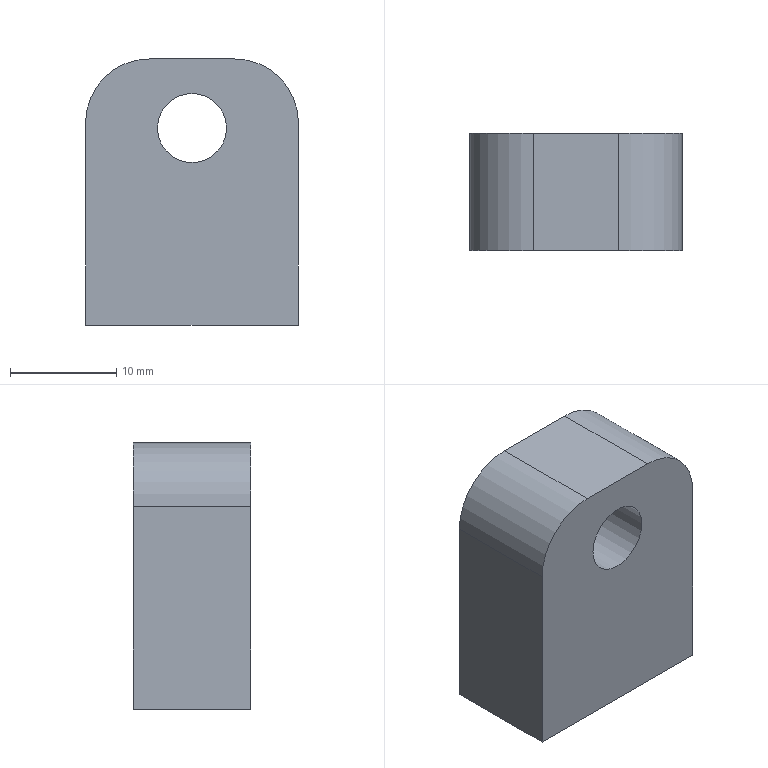Component | NX | SMALL_BRACKET | 1 solid | 13 faces | box 20 x 11 x 25 mm | volume 4714 mm3 | plane 8 | cylinder 5 | commonest cylinder face diameters 12 x2 4 x2 6.5 x1
STEP:
#1=CARTESIAN_POINT('',(0.,0.,0.));
#2=DIRECTION('',(0.,0.,1.));
#3=DIRECTION('',(1.,0.,0.));
#4=AXIS2_PLACEMENT_3D('',#1,#2,#3);
#5=CARTESIAN_POINT('',(9.,19.,36.5));
#6=VERTEX_POINT('',#5);
#7=CARTESIAN_POINT('',(9.,19.,17.5));
#8=VERTEX_POINT('',#7);
#9=CARTESIAN_POINT('',(9.,19.,42.5));
#10=DIRECTION('',(0.,0.,-1.));
#11=VECTOR('',#10,1.);
#12=LINE('',#9,#11);
#13=CARTESIAN_POINT('',(9.,19.,42.5));
#14=DIRECTION('',(1.,0.,0.));
#15=DIRECTION('',(0.,0.,1.));
#16=AXIS2_PLACEMENT_3D('',#13,#14,#15);
#17=PLANE('',#16);
#18=CARTESIAN_POINT('',(0.,0.));
#19=DIRECTION('',(-1.,0.));
#20=VECTOR('',#19,1.);
#21=LINE('',#18,#20);
#22=(GEOMETRIC_REPRESENTATION_CONTEXT(2)PARAMETRIC_REPRESENTATION_CONTEXT()REPRESENTATION_CONTEXT('',''));
#23=DEFINITIONAL_REPRESENTATION('',(#21),#22);
#24=PCURVE('',#17,#23);
#25=CARTESIAN_POINT('',(19.,19.,36.));
#26=DIRECTION('',(0.,-1.,0.));
#27=DIRECTION('',(0.,0.,-1.));
#28=AXIS2_PLACEMENT_3D('',#25,#26,#27);
#29=PLANE('',#28);
#30=CARTESIAN_POINT('',(-6.5,-10.));
#31=DIRECTION('',(1.,0.));
#32=VECTOR('',#31,1.);
#33=LINE('',#30,#32);
#34=(GEOMETRIC_REPRESENTATION_CONTEXT(2)PARAMETRIC_REPRESENTATION_CONTEXT()REPRESENTATION_CONTEXT('',''));
#35=DEFINITIONAL_REPRESENTATION('',(#33),#34);
#36=PCURVE('',#29,#35);
#37=SURFACE_CURVE('',#12,(#24,#36),.PCURVE_S1.);
#38=EDGE_CURVE('',#6,#8,#37,.T.);
#39=ORIENTED_EDGE('',*,*,#38,.F.);
#40=CARTESIAN_POINT('',(9.,30.,36.5));
#41=VERTEX_POINT('',#40);
#42=CARTESIAN_POINT('',(9.,19.,36.5));
#43=DIRECTION('',(0.,1.,0.));
#44=VECTOR('',#43,1.);
#45=LINE('',#42,#44);
#46=CARTESIAN_POINT('',(-6.,0.));
#47=DIRECTION('',(0.,-1.));
#48=VECTOR('',#47,1.);
#49=LINE('',#46,#48);
#50=(GEOMETRIC_REPRESENTATION_CONTEXT(2)PARAMETRIC_REPRESENTATION_CONTEXT()REPRESENTATION_CONTEXT('',''));
#51=DEFINITIONAL_REPRESENTATION('',(#49),#50);
#52=PCURVE('',#17,#51);
#53=CARTESIAN_POINT('',(15.,19.,36.5));
#54=DIRECTION('',(0.,1.,0.));
#55=DIRECTION('',(0.,0.,1.));
#56=AXIS2_PLACEMENT_3D('',#53,#54,#55);
#57=CYLINDRICAL_SURFACE('',#56,6.);
#58=CARTESIAN_POINT('',(4.712,0.));
#59=DIRECTION('',(0.,1.));
#60=VECTOR('',#59,1.);
#61=LINE('',#58,#60);
#62=(GEOMETRIC_REPRESENTATION_CONTEXT(2)PARAMETRIC_REPRESENTATION_CONTEXT()REPRESENTATION_CONTEXT('',''));
#63=DEFINITIONAL_REPRESENTATION('',(#61),#62);
#64=PCURVE('',#57,#63);
#65=SURFACE_CURVE('',#45,(#52,#64),.PCURVE_S1.);
#66=EDGE_CURVE('',#6,#41,#65,.T.);
#67=ORIENTED_EDGE('',*,*,#66,.T.);
#68=CARTESIAN_POINT('',(9.,30.,17.5));
#69=VERTEX_POINT('',#68);
#70=CARTESIAN_POINT('',(9.,30.,42.5));
#71=DIRECTION('',(0.,0.,-1.));
#72=VECTOR('',#71,1.);
#73=LINE('',#70,#72);
#74=CARTESIAN_POINT('',(0.,-11.));
#75=DIRECTION('',(-1.,0.));
#76=VECTOR('',#75,1.);
#77=LINE('',#74,#76);
#78=(GEOMETRIC_REPRESENTATION_CONTEXT(2)PARAMETRIC_REPRESENTATION_CONTEXT()REPRESENTATION_CONTEXT('',''));
#79=DEFINITIONAL_REPRESENTATION('',(#77),#78);
#80=PCURVE('',#17,#79);
#81=CARTESIAN_POINT('',(19.,30.,36.));
#82=DIRECTION('',(0.,-1.,0.));
#83=DIRECTION('',(0.,0.,-1.));
#84=AXIS2_PLACEMENT_3D('',#81,#82,#83);
#85=PLANE('',#84);
#86=CARTESIAN_POINT('',(-6.5,-10.));
#87=DIRECTION('',(1.,0.));
#88=VECTOR('',#87,1.);
#89=LINE('',#86,#88);
#90=(GEOMETRIC_REPRESENTATION_CONTEXT(2)PARAMETRIC_REPRESENTATION_CONTEXT()REPRESENTATION_CONTEXT('',''));
#91=DEFINITIONAL_REPRESENTATION('',(#89),#90);
#92=PCURVE('',#85,#91);
#93=SURFACE_CURVE('',#73,(#80,#92),.PCURVE_S1.);
#94=EDGE_CURVE('',#41,#69,#93,.T.);
#95=ORIENTED_EDGE('',*,*,#94,.T.);
#96=CARTESIAN_POINT('',(9.,19.,17.5));
#97=DIRECTION('',(0.,1.,0.));
#98=VECTOR('',#97,1.);
#99=LINE('',#96,#98);
#100=CARTESIAN_POINT('',(-25.,0.));
#101=DIRECTION('',(0.,-1.));
#102=VECTOR('',#101,1.);
#103=LINE('',#100,#102);
#104=(GEOMETRIC_REPRESENTATION_CONTEXT(2)PARAMETRIC_REPRESENTATION_CONTEXT()REPRESENTATION_CONTEXT('',''));
#105=DEFINITIONAL_REPRESENTATION('',(#103),#104);
#106=PCURVE('',#17,#105);
#107=CARTESIAN_POINT('',(19.,19.,17.5));
#108=DIRECTION('',(0.,0.,1.));
#109=DIRECTION('',(-1.,0.,0.));
#110=AXIS2_PLACEMENT_3D('',#107,#108,#109);
#111=PLANE('',#110);
#112=CARTESIAN_POINT('',(10.,0.));
#113=DIRECTION('',(0.,-1.));
#114=VECTOR('',#113,1.);
#115=LINE('',#112,#114);
#116=(GEOMETRIC_REPRESENTATION_CONTEXT(2)PARAMETRIC_REPRESENTATION_CONTEXT()REPRESENTATION_CONTEXT('',''));
#117=DEFINITIONAL_REPRESENTATION('',(#115),#116);
#118=PCURVE('',#111,#117);
#119=SURFACE_CURVE('',#99,(#106,#118),.PCURVE_S1.);
#120=EDGE_CURVE('',#8,#69,#119,.T.);
#121=ORIENTED_EDGE('',*,*,#120,.F.);
#122=EDGE_LOOP('',(#39,#67,#95,#121));
#123=FACE_BOUND('',#122,.T.);
#124=ADVANCED_FACE('',(#123),#17,.F.);
#125=CARTESIAN_POINT('',(14.5,24.5,17.5));
#126=VERTEX_POINT('',#125);
#127=CARTESIAN_POINT('',(12.5,24.5,17.5));
#128=DIRECTION('',(-0.,0.,-1.));
#129=DIRECTION('',(1.,0.,-0.));
#130=AXIS2_PLACEMENT_3D('',#127,#128,#129);
#131=CIRCLE('',#130,2.);
#132=CARTESIAN_POINT('',(4.5,-5.5));
#133=CARTESIAN_POINT('',(4.5,-2.036));
#134=CARTESIAN_POINT('',(7.5,-3.768));
#135=CARTESIAN_POINT('',(10.5,-5.5));
#136=CARTESIAN_POINT('',(7.5,-7.232));
#137=CARTESIAN_POINT('',(4.5,-8.964));
#138=CARTESIAN_POINT('',(4.5,-5.5));
#139=(BOUNDED_CURVE()B_SPLINE_CURVE(2,(#132,#133,#134,#135,#136,#137,#138),.UNSPECIFIED.,.T.,.F.)B_SPLINE_CURVE_WITH_KNOTS((1,2,2,2,2,1),(-2.094,0.,2.094,4.189,6.283,8.378),.UNSPECIFIED.)CURVE()GEOMETRIC_REPRESENTATION_ITEM()RATIONAL_B_SPLINE_CURVE((1.,0.5,1.,0.5,1.,0.5,1.))REPRESENTATION_ITEM(''));
#140=(GEOMETRIC_REPRESENTATION_CONTEXT(2)PARAMETRIC_REPRESENTATION_CONTEXT()REPRESENTATION_CONTEXT('',''));
#141=DEFINITIONAL_REPRESENTATION('',(#139),#140);
#142=PCURVE('',#111,#141);
#143=CARTESIAN_POINT('',(12.5,24.5,27.5));
#144=DIRECTION('',(-0.,0.,-1.));
#145=DIRECTION('',(1.,0.,-0.));
#146=AXIS2_PLACEMENT_3D('',#143,#144,#145);
#147=CYLINDRICAL_SURFACE('',#146,2.);
#148=CARTESIAN_POINT('',(0.,10.));
#149=DIRECTION('',(1.,0.));
#150=VECTOR('',#149,1.);
#151=LINE('',#148,#150);
#152=(GEOMETRIC_REPRESENTATION_CONTEXT(2)PARAMETRIC_REPRESENTATION_CONTEXT()REPRESENTATION_CONTEXT('',''));
#153=DEFINITIONAL_REPRESENTATION('',(#151),#152);
#154=PCURVE('',#147,#153);
#155=SURFACE_CURVE('',#131,(#142,#154),.PCURVE_S1.);
#156=EDGE_CURVE('',#126,#126,#155,.T.);
#157=ORIENTED_EDGE('',*,*,#156,.F.);
#158=EDGE_LOOP('',(#157));
#159=FACE_BOUND('',#158,.T.);
#160=CARTESIAN_POINT('',(23.5,24.5,17.5));
#161=VERTEX_POINT('',#160);
#162=CARTESIAN_POINT('',(25.5,24.5,17.5));
#163=DIRECTION('',(-0.,0.,-1.));
#164=DIRECTION('',(-1.,0.,0.));
#165=AXIS2_PLACEMENT_3D('',#162,#163,#164);
#166=CIRCLE('',#165,2.);
#167=CARTESIAN_POINT('',(-4.5,-5.5));
#168=CARTESIAN_POINT('',(-4.5,-8.964));
#169=CARTESIAN_POINT('',(-7.5,-7.232));
#170=CARTESIAN_POINT('',(-10.5,-5.5));
#171=CARTESIAN_POINT('',(-7.5,-3.768));
#172=CARTESIAN_POINT('',(-4.5,-2.036));
#173=CARTESIAN_POINT('',(-4.5,-5.5));
#174=(BOUNDED_CURVE()B_SPLINE_CURVE(2,(#167,#168,#169,#170,#171,#172,#173),.UNSPECIFIED.,.T.,.F.)B_SPLINE_CURVE_WITH_KNOTS((1,2,2,2,2,1),(-2.094,0.,2.094,4.189,6.283,8.378),.UNSPECIFIED.)CURVE()GEOMETRIC_REPRESENTATION_ITEM()RATIONAL_B_SPLINE_CURVE((1.,0.5,1.,0.5,1.,0.5,1.))REPRESENTATION_ITEM(''));
#175=(GEOMETRIC_REPRESENTATION_CONTEXT(2)PARAMETRIC_REPRESENTATION_CONTEXT()REPRESENTATION_CONTEXT('',''));
#176=DEFINITIONAL_REPRESENTATION('',(#174),#175);
#177=PCURVE('',#111,#176);
#178=CARTESIAN_POINT('',(25.5,24.5,27.5));
#179=DIRECTION('',(-0.,0.,-1.));
#180=DIRECTION('',(1.,0.,-0.));
#181=AXIS2_PLACEMENT_3D('',#178,#179,#180);
#182=CYLINDRICAL_SURFACE('',#181,2.);
#183=CARTESIAN_POINT('',(3.142,10.));
#184=DIRECTION('',(1.,0.));
#185=VECTOR('',#184,1.);
#186=LINE('',#183,#185);
#187=(GEOMETRIC_REPRESENTATION_CONTEXT(2)PARAMETRIC_REPRESENTATION_CONTEXT()REPRESENTATION_CONTEXT('',''));
#188=DEFINITIONAL_REPRESENTATION('',(#186),#187);
#189=PCURVE('',#182,#188);
#190=SURFACE_CURVE('',#166,(#177,#189),.PCURVE_S1.);
#191=EDGE_CURVE('',#161,#161,#190,.T.);
#192=ORIENTED_EDGE('',*,*,#191,.F.);
#193=EDGE_LOOP('',(#192));
#194=FACE_BOUND('',#193,.T.);
#195=CARTESIAN_POINT('',(29.,30.,17.5));
#196=VERTEX_POINT('',#195);
#197=CARTESIAN_POINT('',(19.,30.,17.5));
#198=DIRECTION('',(1.,0.,-0.));
#199=VECTOR('',#198,1.);
#200=LINE('',#197,#199);
#201=CARTESIAN_POINT('',(0.,-11.));
#202=DIRECTION('',(-1.,0.));
#203=VECTOR('',#202,1.);
#204=LINE('',#201,#203);
#205=(GEOMETRIC_REPRESENTATION_CONTEXT(2)PARAMETRIC_REPRESENTATION_CONTEXT()REPRESENTATION_CONTEXT('',''));
#206=DEFINITIONAL_REPRESENTATION('',(#204),#205);
#207=PCURVE('',#111,#206);
#208=CARTESIAN_POINT('',(18.5,0.));
#209=DIRECTION('',(0.,1.));
#210=VECTOR('',#209,1.);
#211=LINE('',#208,#210);
#212=(GEOMETRIC_REPRESENTATION_CONTEXT(2)PARAMETRIC_REPRESENTATION_CONTEXT()REPRESENTATION_CONTEXT('',''));
#213=DEFINITIONAL_REPRESENTATION('',(#211),#212);
#214=PCURVE('',#85,#213);
#215=SURFACE_CURVE('',#200,(#207,#214),.PCURVE_S1.);
#216=EDGE_CURVE('',#69,#196,#215,.T.);
#217=ORIENTED_EDGE('',*,*,#216,.T.);
#218=CARTESIAN_POINT('',(29.,19.,17.5));
#219=VERTEX_POINT('',#218);
#220=CARTESIAN_POINT('',(29.,19.,17.5));
#221=DIRECTION('',(0.,1.,0.));
#222=VECTOR('',#221,1.);
#223=LINE('',#220,#222);
#224=CARTESIAN_POINT('',(-10.,0.));
#225=DIRECTION('',(0.,-1.));
#226=VECTOR('',#225,1.);
#227=LINE('',#224,#226);
#228=(GEOMETRIC_REPRESENTATION_CONTEXT(2)PARAMETRIC_REPRESENTATION_CONTEXT()REPRESENTATION_CONTEXT('',''));
#229=DEFINITIONAL_REPRESENTATION('',(#227),#228);
#230=PCURVE('',#111,#229);
#231=CARTESIAN_POINT('',(29.,19.,17.5));
#232=DIRECTION('',(-1.,0.,0.));
#233=DIRECTION('',(0.,0.,-1.));
#234=AXIS2_PLACEMENT_3D('',#231,#232,#233);
#235=PLANE('',#234);
#236=CARTESIAN_POINT('',(0.,0.));
#237=DIRECTION('',(0.,-1.));
#238=VECTOR('',#237,1.);
#239=LINE('',#236,#238);
#240=(GEOMETRIC_REPRESENTATION_CONTEXT(2)PARAMETRIC_REPRESENTATION_CONTEXT()REPRESENTATION_CONTEXT('',''));
#241=DEFINITIONAL_REPRESENTATION('',(#239),#240);
#242=PCURVE('',#235,#241);
#243=SURFACE_CURVE('',#223,(#230,#242),.PCURVE_S1.);
#244=EDGE_CURVE('',#219,#196,#243,.T.);
#245=ORIENTED_EDGE('',*,*,#244,.F.);
#246=CARTESIAN_POINT('',(9.,19.,17.5));
#247=DIRECTION('',(1.,0.,0.));
#248=VECTOR('',#247,1.);
#249=LINE('',#246,#248);
#250=CARTESIAN_POINT('',(10.,0.));
#251=DIRECTION('',(-1.,0.));
#252=VECTOR('',#251,1.);
#253=LINE('',#250,#252);
#254=(GEOMETRIC_REPRESENTATION_CONTEXT(2)PARAMETRIC_REPRESENTATION_CONTEXT()REPRESENTATION_CONTEXT('',''));
#255=DEFINITIONAL_REPRESENTATION('',(#253),#254);
#256=PCURVE('',#111,#255);
#257=CARTESIAN_POINT('',(18.5,-10.));
#258=DIRECTION('',(-0.,1.));
#259=VECTOR('',#258,1.);
#260=LINE('',#257,#259);
#261=(GEOMETRIC_REPRESENTATION_CONTEXT(2)PARAMETRIC_REPRESENTATION_CONTEXT()REPRESENTATION_CONTEXT('',''));
#262=DEFINITIONAL_REPRESENTATION('',(#260),#261);
#263=PCURVE('',#29,#262);
#264=SURFACE_CURVE('',#249,(#256,#263),.PCURVE_S1.);
#265=EDGE_CURVE('',#8,#219,#264,.T.);
#266=ORIENTED_EDGE('',*,*,#265,.F.);
#267=ORIENTED_EDGE('',*,*,#120,.T.);
#268=EDGE_LOOP('',(#217,#245,#266,#267));
#269=FACE_BOUND('',#268,.T.);
#270=ADVANCED_FACE('',(#159,#194,#269),#111,.F.);
#271=CARTESIAN_POINT('',(29.,30.,36.5));
#272=VERTEX_POINT('',#271);
#273=CARTESIAN_POINT('',(29.,30.,17.5));
#274=DIRECTION('',(0.,0.,1.));
#275=VECTOR('',#274,1.);
#276=LINE('',#273,#275);
#277=CARTESIAN_POINT('',(0.,-11.));
#278=DIRECTION('',(-1.,0.));
#279=VECTOR('',#278,1.);
#280=LINE('',#277,#279);
#281=(GEOMETRIC_REPRESENTATION_CONTEXT(2)PARAMETRIC_REPRESENTATION_CONTEXT()REPRESENTATION_CONTEXT('',''));
#282=DEFINITIONAL_REPRESENTATION('',(#280),#281);
#283=PCURVE('',#235,#282);
#284=CARTESIAN_POINT('',(18.5,10.));
#285=DIRECTION('',(-1.,0.));
#286=VECTOR('',#285,1.);
#287=LINE('',#284,#286);
#288=(GEOMETRIC_REPRESENTATION_CONTEXT(2)PARAMETRIC_REPRESENTATION_CONTEXT()REPRESENTATION_CONTEXT('',''));
#289=DEFINITIONAL_REPRESENTATION('',(#287),#288);
#290=PCURVE('',#85,#289);
#291=SURFACE_CURVE('',#276,(#283,#290),.PCURVE_S1.);
#292=EDGE_CURVE('',#196,#272,#291,.T.);
#293=ORIENTED_EDGE('',*,*,#292,.T.);
#294=CARTESIAN_POINT('',(29.,19.,36.5));
#295=VERTEX_POINT('',#294);
#296=CARTESIAN_POINT('',(29.,19.,36.5));
#297=DIRECTION('',(0.,-1.,0.));
#298=VECTOR('',#297,1.);
#299=LINE('',#296,#298);
#300=CARTESIAN_POINT('',(-19.,0.));
#301=DIRECTION('',(0.,1.));
#302=VECTOR('',#301,1.);
#303=LINE('',#300,#302);
#304=(GEOMETRIC_REPRESENTATION_CONTEXT(2)PARAMETRIC_REPRESENTATION_CONTEXT()REPRESENTATION_CONTEXT('',''));
#305=DEFINITIONAL_REPRESENTATION('',(#303),#304);
#306=PCURVE('',#235,#305);
#307=CARTESIAN_POINT('',(23.,19.,36.5));
#308=DIRECTION('',(0.,1.,0.));
#309=DIRECTION('',(0.,0.,1.));
#310=AXIS2_PLACEMENT_3D('',#307,#308,#309);
#311=CYLINDRICAL_SURFACE('',#310,6.);
#312=CARTESIAN_POINT('',(1.571,0.));
#313=DIRECTION('',(0.,-1.));
#314=VECTOR('',#313,1.);
#315=LINE('',#312,#314);
#316=(GEOMETRIC_REPRESENTATION_CONTEXT(2)PARAMETRIC_REPRESENTATION_CONTEXT()REPRESENTATION_CONTEXT('',''));
#317=DEFINITIONAL_REPRESENTATION('',(#315),#316);
#318=PCURVE('',#311,#317);
#319=SURFACE_CURVE('',#299,(#306,#318),.PCURVE_S1.);
#320=EDGE_CURVE('',#272,#295,#319,.T.);
#321=ORIENTED_EDGE('',*,*,#320,.T.);
#322=CARTESIAN_POINT('',(29.,19.,17.5));
#323=DIRECTION('',(0.,0.,1.));
#324=VECTOR('',#323,1.);
#325=LINE('',#322,#324);
#326=CARTESIAN_POINT('',(0.,0.));
#327=DIRECTION('',(-1.,0.));
#328=VECTOR('',#327,1.);
#329=LINE('',#326,#328);
#330=(GEOMETRIC_REPRESENTATION_CONTEXT(2)PARAMETRIC_REPRESENTATION_CONTEXT()REPRESENTATION_CONTEXT('',''));
#331=DEFINITIONAL_REPRESENTATION('',(#329),#330);
#332=PCURVE('',#235,#331);
#333=CARTESIAN_POINT('',(18.5,10.));
#334=DIRECTION('',(-1.,0.));
#335=VECTOR('',#334,1.);
#336=LINE('',#333,#335);
#337=(GEOMETRIC_REPRESENTATION_CONTEXT(2)PARAMETRIC_REPRESENTATION_CONTEXT()REPRESENTATION_CONTEXT('',''));
#338=DEFINITIONAL_REPRESENTATION('',(#336),#337);
#339=PCURVE('',#29,#338);
#340=SURFACE_CURVE('',#325,(#332,#339),.PCURVE_S1.);
#341=EDGE_CURVE('',#219,#295,#340,.T.);
#342=ORIENTED_EDGE('',*,*,#341,.F.);
#343=ORIENTED_EDGE('',*,*,#244,.T.);
#344=EDGE_LOOP('',(#293,#321,#342,#343));
#345=FACE_BOUND('',#344,.T.);
#346=ADVANCED_FACE('',(#345),#235,.F.);
#347=CARTESIAN_POINT('',(23.,19.,42.5));
#348=VERTEX_POINT('',#347);
#349=CARTESIAN_POINT('',(15.,19.,42.5));
#350=VERTEX_POINT('',#349);
#351=CARTESIAN_POINT('',(29.,19.,42.5));
#352=DIRECTION('',(-1.,0.,0.));
#353=VECTOR('',#352,1.);
#354=LINE('',#351,#353);
#355=CARTESIAN_POINT('',(19.,19.,42.5));
#356=DIRECTION('',(0.,0.,-1.));
#357=DIRECTION('',(1.,0.,0.));
#358=AXIS2_PLACEMENT_3D('',#355,#356,#357);
#359=PLANE('',#358);
#360=CARTESIAN_POINT('',(10.,0.));
#361=DIRECTION('',(-1.,0.));
#362=VECTOR('',#361,1.);
#363=LINE('',#360,#362);
#364=(GEOMETRIC_REPRESENTATION_CONTEXT(2)PARAMETRIC_REPRESENTATION_CONTEXT()REPRESENTATION_CONTEXT('',''));
#365=DEFINITIONAL_REPRESENTATION('',(#363),#364);
#366=PCURVE('',#359,#365);
#367=CARTESIAN_POINT('',(-6.5,10.));
#368=DIRECTION('',(-0.,-1.));
#369=VECTOR('',#368,1.);
#370=LINE('',#367,#369);
#371=(GEOMETRIC_REPRESENTATION_CONTEXT(2)PARAMETRIC_REPRESENTATION_CONTEXT()REPRESENTATION_CONTEXT('',''));
#372=DEFINITIONAL_REPRESENTATION('',(#370),#371);
#373=PCURVE('',#29,#372);
#374=SURFACE_CURVE('',#354,(#366,#373),.PCURVE_S1.);
#375=EDGE_CURVE('',#348,#350,#374,.T.);
#376=ORIENTED_EDGE('',*,*,#375,.F.);
#377=CARTESIAN_POINT('',(23.,30.,42.5));
#378=VERTEX_POINT('',#377);
#379=CARTESIAN_POINT('',(23.,19.,42.5));
#380=DIRECTION('',(0.,1.,0.));
#381=VECTOR('',#380,1.);
#382=LINE('',#379,#381);
#383=CARTESIAN_POINT('',(4.,0.));
#384=DIRECTION('',(0.,-1.));
#385=VECTOR('',#384,1.);
#386=LINE('',#383,#385);
#387=(GEOMETRIC_REPRESENTATION_CONTEXT(2)PARAMETRIC_REPRESENTATION_CONTEXT()REPRESENTATION_CONTEXT('',''));
#388=DEFINITIONAL_REPRESENTATION('',(#386),#387);
#389=PCURVE('',#359,#388);
#390=CARTESIAN_POINT('',(0.,0.));
#391=DIRECTION('',(0.,1.));
#392=VECTOR('',#391,1.);
#393=LINE('',#390,#392);
#394=(GEOMETRIC_REPRESENTATION_CONTEXT(2)PARAMETRIC_REPRESENTATION_CONTEXT()REPRESENTATION_CONTEXT('',''));
#395=DEFINITIONAL_REPRESENTATION('',(#393),#394);
#396=PCURVE('',#311,#395);
#397=SURFACE_CURVE('',#382,(#389,#396),.PCURVE_S1.);
#398=EDGE_CURVE('',#348,#378,#397,.T.);
#399=ORIENTED_EDGE('',*,*,#398,.T.);
#400=CARTESIAN_POINT('',(15.,30.,42.5));
#401=VERTEX_POINT('',#400);
#402=CARTESIAN_POINT('',(19.,30.,42.5));
#403=DIRECTION('',(-1.,0.,-0.));
#404=VECTOR('',#403,1.);
#405=LINE('',#402,#404);
#406=CARTESIAN_POINT('',(0.,-11.));
#407=DIRECTION('',(-1.,0.));
#408=VECTOR('',#407,1.);
#409=LINE('',#406,#408);
#410=(GEOMETRIC_REPRESENTATION_CONTEXT(2)PARAMETRIC_REPRESENTATION_CONTEXT()REPRESENTATION_CONTEXT('',''));
#411=DEFINITIONAL_REPRESENTATION('',(#409),#410);
#412=PCURVE('',#359,#411);
#413=CARTESIAN_POINT('',(-6.5,0.));
#414=DIRECTION('',(0.,-1.));
#415=VECTOR('',#414,1.);
#416=LINE('',#413,#415);
#417=(GEOMETRIC_REPRESENTATION_CONTEXT(2)PARAMETRIC_REPRESENTATION_CONTEXT()REPRESENTATION_CONTEXT('',''));
#418=DEFINITIONAL_REPRESENTATION('',(#416),#417);
#419=PCURVE('',#85,#418);
#420=SURFACE_CURVE('',#405,(#412,#419),.PCURVE_S1.);
#421=EDGE_CURVE('',#378,#401,#420,.T.);
#422=ORIENTED_EDGE('',*,*,#421,.T.);
#423=CARTESIAN_POINT('',(15.,19.,42.5));
#424=DIRECTION('',(0.,-1.,0.));
#425=VECTOR('',#424,1.);
#426=LINE('',#423,#425);
#427=CARTESIAN_POINT('',(-4.,0.));
#428=DIRECTION('',(0.,1.));
#429=VECTOR('',#428,1.);
#430=LINE('',#427,#429);
#431=(GEOMETRIC_REPRESENTATION_CONTEXT(2)PARAMETRIC_REPRESENTATION_CONTEXT()REPRESENTATION_CONTEXT('',''));
#432=DEFINITIONAL_REPRESENTATION('',(#430),#431);
#433=PCURVE('',#359,#432);
#434=CARTESIAN_POINT('',(6.283,0.));
#435=DIRECTION('',(0.,-1.));
#436=VECTOR('',#435,1.);
#437=LINE('',#434,#436);
#438=(GEOMETRIC_REPRESENTATION_CONTEXT(2)PARAMETRIC_REPRESENTATION_CONTEXT()REPRESENTATION_CONTEXT('',''));
#439=DEFINITIONAL_REPRESENTATION('',(#437),#438);
#440=PCURVE('',#57,#439);
#441=SURFACE_CURVE('',#426,(#433,#440),.PCURVE_S1.);
#442=EDGE_CURVE('',#401,#350,#441,.T.);
#443=ORIENTED_EDGE('',*,*,#442,.T.);
#444=EDGE_LOOP('',(#376,#399,#422,#443));
#445=FACE_BOUND('',#444,.T.);
#446=ADVANCED_FACE('',(#445),#359,.F.);
#447=CARTESIAN_POINT('',(22.25,19.,36.));
#448=VERTEX_POINT('',#447);
#449=CARTESIAN_POINT('',(19.,19.,36.));
#450=DIRECTION('',(0.,-1.,0.));
#451=DIRECTION('',(1.,0.,0.));
#452=AXIS2_PLACEMENT_3D('',#449,#450,#451);
#453=CIRCLE('',#452,3.25);
#454=CARTESIAN_POINT('',(19.,19.,36.));
#455=DIRECTION('',(0.,1.,0.));
#456=DIRECTION('',(0.,0.,1.));
#457=AXIS2_PLACEMENT_3D('',#454,#455,#456);
#458=CYLINDRICAL_SURFACE('',#457,3.25);
#459=CARTESIAN_POINT('',(7.854,0.));
#460=DIRECTION('',(-1.,0.));
#461=VECTOR('',#460,1.);
#462=LINE('',#459,#461);
#463=(GEOMETRIC_REPRESENTATION_CONTEXT(2)PARAMETRIC_REPRESENTATION_CONTEXT()REPRESENTATION_CONTEXT('',''));
#464=DEFINITIONAL_REPRESENTATION('',(#462),#463);
#465=PCURVE('',#458,#464);
#466=CARTESIAN_POINT('',(0.,0.));
#467=DIRECTION('',(0.,1.));
#468=AXIS2_PLACEMENT_2D('',#466,#467);
#469=CIRCLE('',#468,3.25);
#470=(GEOMETRIC_REPRESENTATION_CONTEXT(2)PARAMETRIC_REPRESENTATION_CONTEXT()REPRESENTATION_CONTEXT('',''));
#471=DEFINITIONAL_REPRESENTATION('',(#469),#470);
#472=PCURVE('',#29,#471);
#473=SURFACE_CURVE('',#453,(#465,#472),.PCURVE_S1.);
#474=EDGE_CURVE('',#448,#448,#473,.T.);
#475=ORIENTED_EDGE('',*,*,#474,.F.);
#476=CARTESIAN_POINT('',(22.25,30.,36.));
#477=VERTEX_POINT('',#476);
#478=CARTESIAN_POINT('',(22.25,19.,36.));
#479=CARTESIAN_POINT('',(22.25,30.,36.));
#480=B_SPLINE_CURVE_WITH_KNOTS('',1,(#478,#479),.UNSPECIFIED.,.F.,.F.,(2,2),(0.,11.),.PIECEWISE_BEZIER_KNOTS.);
#481=CARTESIAN_POINT('',(7.854,0.));
#482=DIRECTION('',(0.,1.));
#483=VECTOR('',#482,1.);
#484=LINE('',#481,#483);
#485=(GEOMETRIC_REPRESENTATION_CONTEXT(2)PARAMETRIC_REPRESENTATION_CONTEXT()REPRESENTATION_CONTEXT('',''));
#486=DEFINITIONAL_REPRESENTATION('',(#484),#485);
#487=PCURVE('',#458,#486);
#488=CARTESIAN_POINT('',(1.571,0.));
#489=DIRECTION('',(0.,1.));
#490=VECTOR('',#489,1.);
#491=LINE('',#488,#490);
#492=(GEOMETRIC_REPRESENTATION_CONTEXT(2)PARAMETRIC_REPRESENTATION_CONTEXT()REPRESENTATION_CONTEXT('',''));
#493=DEFINITIONAL_REPRESENTATION('',(#491),#492);
#494=PCURVE('',#458,#493);
#495=SEAM_CURVE('',#480,(#487,#494),.PCURVE_S1.);
#496=EDGE_CURVE('',#448,#477,#495,.T.);
#497=ORIENTED_EDGE('',*,*,#496,.T.);
#498=CARTESIAN_POINT('',(19.,30.,36.));
#499=DIRECTION('',(0.,-1.,0.));
#500=DIRECTION('',(1.,0.,0.));
#501=AXIS2_PLACEMENT_3D('',#498,#499,#500);
#502=CIRCLE('',#501,3.25);
#503=CARTESIAN_POINT('',(7.854,11.));
#504=DIRECTION('',(-1.,0.));
#505=VECTOR('',#504,1.);
#506=LINE('',#503,#505);
#507=(GEOMETRIC_REPRESENTATION_CONTEXT(2)PARAMETRIC_REPRESENTATION_CONTEXT()REPRESENTATION_CONTEXT('',''));
#508=DEFINITIONAL_REPRESENTATION('',(#506),#507);
#509=PCURVE('',#458,#508);
#510=CARTESIAN_POINT('',(0.,0.));
#511=DIRECTION('',(0.,1.));
#512=AXIS2_PLACEMENT_2D('',#510,#511);
#513=CIRCLE('',#512,3.25);
#514=(GEOMETRIC_REPRESENTATION_CONTEXT(2)PARAMETRIC_REPRESENTATION_CONTEXT()REPRESENTATION_CONTEXT('',''));
#515=DEFINITIONAL_REPRESENTATION('',(#513),#514);
#516=PCURVE('',#85,#515);
#517=SURFACE_CURVE('',#502,(#509,#516),.PCURVE_S1.);
#518=EDGE_CURVE('',#477,#477,#517,.T.);
#519=ORIENTED_EDGE('',*,*,#518,.T.);
#520=ORIENTED_EDGE('',*,*,#496,.F.);
#521=EDGE_LOOP('',(#475,#497,#519,#520));
#522=FACE_BOUND('',#521,.F.);
#523=ADVANCED_FACE('',(#522),#458,.F.);
#524=ORIENTED_EDGE('',*,*,#341,.T.);
#525=CARTESIAN_POINT('',(23.,19.,36.5));
#526=DIRECTION('',(0.,-1.,0.));
#527=DIRECTION('',(0.,0.,-1.));
#528=AXIS2_PLACEMENT_3D('',#525,#526,#527);
#529=CIRCLE('',#528,6.);
#530=CARTESIAN_POINT('',(-0.5,4.));
#531=DIRECTION('',(1.,0.));
#532=AXIS2_PLACEMENT_2D('',#530,#531);
#533=CIRCLE('',#532,6.);
#534=(GEOMETRIC_REPRESENTATION_CONTEXT(2)PARAMETRIC_REPRESENTATION_CONTEXT()REPRESENTATION_CONTEXT('',''));
#535=DEFINITIONAL_REPRESENTATION('',(#533),#534);
#536=PCURVE('',#29,#535);
#537=CARTESIAN_POINT('',(3.142,0.));
#538=DIRECTION('',(-1.,0.));
#539=VECTOR('',#538,1.);
#540=LINE('',#537,#539);
#541=(GEOMETRIC_REPRESENTATION_CONTEXT(2)PARAMETRIC_REPRESENTATION_CONTEXT()REPRESENTATION_CONTEXT('',''));
#542=DEFINITIONAL_REPRESENTATION('',(#540),#541);
#543=PCURVE('',#311,#542);
#544=SURFACE_CURVE('',#529,(#536,#543),.PCURVE_S1.);
#545=EDGE_CURVE('',#295,#348,#544,.T.);
#546=ORIENTED_EDGE('',*,*,#545,.T.);
#547=ORIENTED_EDGE('',*,*,#375,.T.);
#548=CARTESIAN_POINT('',(15.,19.,36.5));
#549=DIRECTION('',(0.,-1.,0.));
#550=DIRECTION('',(0.,0.,-1.));
#551=AXIS2_PLACEMENT_3D('',#548,#549,#550);
#552=CIRCLE('',#551,6.);
#553=CARTESIAN_POINT('',(-0.5,-4.));
#554=DIRECTION('',(1.,0.));
#555=AXIS2_PLACEMENT_2D('',#553,#554);
#556=CIRCLE('',#555,6.);
#557=(GEOMETRIC_REPRESENTATION_CONTEXT(2)PARAMETRIC_REPRESENTATION_CONTEXT()REPRESENTATION_CONTEXT('',''));
#558=DEFINITIONAL_REPRESENTATION('',(#556),#557);
#559=PCURVE('',#29,#558);
#560=CARTESIAN_POINT('',(9.425,0.));
#561=DIRECTION('',(-1.,0.));
#562=VECTOR('',#561,1.);
#563=LINE('',#560,#562);
#564=(GEOMETRIC_REPRESENTATION_CONTEXT(2)PARAMETRIC_REPRESENTATION_CONTEXT()REPRESENTATION_CONTEXT('',''));
#565=DEFINITIONAL_REPRESENTATION('',(#563),#564);
#566=PCURVE('',#57,#565);
#567=SURFACE_CURVE('',#552,(#559,#566),.PCURVE_S1.);
#568=EDGE_CURVE('',#350,#6,#567,.T.);
#569=ORIENTED_EDGE('',*,*,#568,.T.);
#570=ORIENTED_EDGE('',*,*,#38,.T.);
#571=ORIENTED_EDGE('',*,*,#265,.T.);
#572=EDGE_LOOP('',(#524,#546,#547,#569,#570,#571));
#573=FACE_BOUND('',#572,.T.);
#574=ORIENTED_EDGE('',*,*,#474,.F.);
#575=EDGE_LOOP('',(#574));
#576=FACE_BOUND('',#575,.T.);
#577=ADVANCED_FACE('',(#573,#576),#29,.T.);
#578=ORIENTED_EDGE('',*,*,#421,.F.);
#579=CARTESIAN_POINT('',(23.,30.,36.5));
#580=DIRECTION('',(0.,1.,0.));
#581=DIRECTION('',(0.,0.,-1.));
#582=AXIS2_PLACEMENT_3D('',#579,#580,#581);
#583=CIRCLE('',#582,6.);
#584=CARTESIAN_POINT('',(5.5,4.));
#585=CARTESIAN_POINT('',(5.5,-6.392));
#586=CARTESIAN_POINT('',(-3.5,-1.196));
#587=CARTESIAN_POINT('',(-12.5,4.));
#588=CARTESIAN_POINT('',(-3.5,9.196));
#589=CARTESIAN_POINT('',(5.5,14.392));
#590=CARTESIAN_POINT('',(5.5,4.));
#591=(BOUNDED_CURVE()B_SPLINE_CURVE(2,(#584,#585,#586,#587,#588,#589,#590),.UNSPECIFIED.,.T.,.F.)B_SPLINE_CURVE_WITH_KNOTS((1,2,2,2,2,1),(-2.094,0.,2.094,4.189,6.283,8.378),.UNSPECIFIED.)CURVE()GEOMETRIC_REPRESENTATION_ITEM()RATIONAL_B_SPLINE_CURVE((1.,0.5,1.,0.5,1.,0.5,1.))REPRESENTATION_ITEM(''));
#592=(GEOMETRIC_REPRESENTATION_CONTEXT(2)PARAMETRIC_REPRESENTATION_CONTEXT()REPRESENTATION_CONTEXT('',''));
#593=DEFINITIONAL_REPRESENTATION('',(#591),#592);
#594=PCURVE('',#85,#593);
#595=CARTESIAN_POINT('',(-3.142,11.));
#596=DIRECTION('',(1.,0.));
#597=VECTOR('',#596,1.);
#598=LINE('',#595,#597);
#599=(GEOMETRIC_REPRESENTATION_CONTEXT(2)PARAMETRIC_REPRESENTATION_CONTEXT()REPRESENTATION_CONTEXT('',''));
#600=DEFINITIONAL_REPRESENTATION('',(#598),#599);
#601=PCURVE('',#311,#600);
#602=SURFACE_CURVE('',#583,(#594,#601),.PCURVE_S1.);
#603=EDGE_CURVE('',#378,#272,#602,.T.);
#604=ORIENTED_EDGE('',*,*,#603,.T.);
#605=ORIENTED_EDGE('',*,*,#292,.F.);
#606=ORIENTED_EDGE('',*,*,#216,.F.);
#607=ORIENTED_EDGE('',*,*,#94,.F.);
#608=CARTESIAN_POINT('',(15.,30.,36.5));
#609=DIRECTION('',(0.,1.,0.));
#610=DIRECTION('',(0.,0.,-1.));
#611=AXIS2_PLACEMENT_3D('',#608,#609,#610);
#612=CIRCLE('',#611,6.);
#613=CARTESIAN_POINT('',(5.5,-4.));
#614=CARTESIAN_POINT('',(5.5,-14.392));
#615=CARTESIAN_POINT('',(-3.5,-9.196));
#616=CARTESIAN_POINT('',(-12.5,-4.));
#617=CARTESIAN_POINT('',(-3.5,1.196));
#618=CARTESIAN_POINT('',(5.5,6.392));
#619=CARTESIAN_POINT('',(5.5,-4.));
#620=(BOUNDED_CURVE()B_SPLINE_CURVE(2,(#613,#614,#615,#616,#617,#618,#619),.UNSPECIFIED.,.T.,.F.)B_SPLINE_CURVE_WITH_KNOTS((1,2,2,2,2,1),(-2.094,0.,2.094,4.189,6.283,8.378),.UNSPECIFIED.)CURVE()GEOMETRIC_REPRESENTATION_ITEM()RATIONAL_B_SPLINE_CURVE((1.,0.5,1.,0.5,1.,0.5,1.))REPRESENTATION_ITEM(''));
#621=(GEOMETRIC_REPRESENTATION_CONTEXT(2)PARAMETRIC_REPRESENTATION_CONTEXT()REPRESENTATION_CONTEXT('',''));
#622=DEFINITIONAL_REPRESENTATION('',(#620),#621);
#623=PCURVE('',#85,#622);
#624=CARTESIAN_POINT('',(3.142,11.));
#625=DIRECTION('',(1.,0.));
#626=VECTOR('',#625,1.);
#627=LINE('',#624,#626);
#628=(GEOMETRIC_REPRESENTATION_CONTEXT(2)PARAMETRIC_REPRESENTATION_CONTEXT()REPRESENTATION_CONTEXT('',''));
#629=DEFINITIONAL_REPRESENTATION('',(#627),#628);
#630=PCURVE('',#57,#629);
#631=SURFACE_CURVE('',#612,(#623,#630),.PCURVE_S1.);
#632=EDGE_CURVE('',#41,#401,#631,.T.);
#633=ORIENTED_EDGE('',*,*,#632,.T.);
#634=EDGE_LOOP('',(#578,#604,#605,#606,#607,#633));
#635=FACE_BOUND('',#634,.T.);
#636=ORIENTED_EDGE('',*,*,#518,.T.);
#637=EDGE_LOOP('',(#636));
#638=FACE_BOUND('',#637,.T.);
#639=ADVANCED_FACE('',(#635,#638),#85,.F.);
#640=ORIENTED_EDGE('',*,*,#545,.F.);
#641=ORIENTED_EDGE('',*,*,#320,.F.);
#642=ORIENTED_EDGE('',*,*,#603,.F.);
#643=ORIENTED_EDGE('',*,*,#398,.F.);
#644=EDGE_LOOP('',(#640,#641,#642,#643));
#645=FACE_BOUND('',#644,.T.);
#646=ADVANCED_FACE('',(#645),#311,.T.);
#647=ORIENTED_EDGE('',*,*,#568,.F.);
#648=ORIENTED_EDGE('',*,*,#442,.F.);
#649=ORIENTED_EDGE('',*,*,#632,.F.);
#650=ORIENTED_EDGE('',*,*,#66,.F.);
#651=EDGE_LOOP('',(#647,#648,#649,#650));
#652=FACE_BOUND('',#651,.T.);
#653=ADVANCED_FACE('',(#652),#57,.T.);
#654=CARTESIAN_POINT('',(23.5,24.5,27.5));
#655=VERTEX_POINT('',#654);
#656=CARTESIAN_POINT('',(25.5,24.5,27.5));
#657=DIRECTION('',(0.,0.,1.));
#658=DIRECTION('',(-1.,0.,0.));
#659=AXIS2_PLACEMENT_3D('',#656,#657,#658);
#660=CIRCLE('',#659,2.);
#661=CARTESIAN_POINT('',(9.425,0.));
#662=DIRECTION('',(-1.,0.));
#663=VECTOR('',#662,1.);
#664=LINE('',#661,#663);
#665=(GEOMETRIC_REPRESENTATION_CONTEXT(2)PARAMETRIC_REPRESENTATION_CONTEXT()REPRESENTATION_CONTEXT('',''));
#666=DEFINITIONAL_REPRESENTATION('',(#664),#665);
#667=PCURVE('',#182,#666);
#668=CARTESIAN_POINT('',(25.5,24.5,27.5));
#669=DIRECTION('',(-0.,0.,-1.));
#670=DIRECTION('',(1.,0.,-0.));
#671=AXIS2_PLACEMENT_3D('',#668,#669,#670);
#672=PLANE('',#671);
#673=CARTESIAN_POINT('',(-2.,0.));
#674=CARTESIAN_POINT('',(-2.,3.464));
#675=CARTESIAN_POINT('',(1.,1.732));
#676=CARTESIAN_POINT('',(4.,0.));
#677=CARTESIAN_POINT('',(1.,-1.732));
#678=CARTESIAN_POINT('',(-2.,-3.464));
#679=CARTESIAN_POINT('',(-2.,0.));
#680=(BOUNDED_CURVE()B_SPLINE_CURVE(2,(#673,#674,#675,#676,#677,#678,#679),.UNSPECIFIED.,.T.,.F.)B_SPLINE_CURVE_WITH_KNOTS((1,2,2,2,2,1),(-2.094,0.,2.094,4.189,6.283,8.378),.UNSPECIFIED.)CURVE()GEOMETRIC_REPRESENTATION_ITEM()RATIONAL_B_SPLINE_CURVE((1.,0.5,1.,0.5,1.,0.5,1.))REPRESENTATION_ITEM(''));
#681=(GEOMETRIC_REPRESENTATION_CONTEXT(2)PARAMETRIC_REPRESENTATION_CONTEXT()REPRESENTATION_CONTEXT('',''));
#682=DEFINITIONAL_REPRESENTATION('',(#680),#681);
#683=PCURVE('',#672,#682);
#684=SURFACE_CURVE('',#660,(#667,#683),.PCURVE_S1.);
#685=EDGE_CURVE('',#655,#655,#684,.T.);
#686=ORIENTED_EDGE('',*,*,#685,.F.);
#687=CARTESIAN_POINT('',(23.5,24.5,27.5));
#688=CARTESIAN_POINT('',(23.5,24.5,17.5));
#689=B_SPLINE_CURVE_WITH_KNOTS('',1,(#687,#688),.UNSPECIFIED.,.F.,.F.,(2,2),(0.,10.),.PIECEWISE_BEZIER_KNOTS.);
#690=CARTESIAN_POINT('',(9.425,0.));
#691=DIRECTION('',(0.,1.));
#692=VECTOR('',#691,1.);
#693=LINE('',#690,#692);
#694=(GEOMETRIC_REPRESENTATION_CONTEXT(2)PARAMETRIC_REPRESENTATION_CONTEXT()REPRESENTATION_CONTEXT('',''));
#695=DEFINITIONAL_REPRESENTATION('',(#693),#694);
#696=PCURVE('',#182,#695);
#697=CARTESIAN_POINT('',(3.142,0.));
#698=DIRECTION('',(0.,1.));
#699=VECTOR('',#698,1.);
#700=LINE('',#697,#699);
#701=(GEOMETRIC_REPRESENTATION_CONTEXT(2)PARAMETRIC_REPRESENTATION_CONTEXT()REPRESENTATION_CONTEXT('',''));
#702=DEFINITIONAL_REPRESENTATION('',(#700),#701);
#703=PCURVE('',#182,#702);
#704=SEAM_CURVE('',#689,(#696,#703),.PCURVE_S1.);
#705=EDGE_CURVE('',#655,#161,#704,.T.);
#706=ORIENTED_EDGE('',*,*,#705,.T.);
#707=ORIENTED_EDGE('',*,*,#191,.F.);
#708=ORIENTED_EDGE('',*,*,#705,.F.);
#709=EDGE_LOOP('',(#686,#706,#707,#708));
#710=FACE_BOUND('',#709,.F.);
#711=ADVANCED_FACE('',(#710),#182,.F.);
#712=ORIENTED_EDGE('',*,*,#685,.F.);
#713=EDGE_LOOP('',(#712));
#714=FACE_BOUND('',#713,.T.);
#715=ADVANCED_FACE('',(#714),#672,.T.);
#716=CARTESIAN_POINT('',(14.5,24.5,27.5));
#717=VERTEX_POINT('',#716);
#718=CARTESIAN_POINT('',(12.5,24.5,27.5));
#719=DIRECTION('',(0.,0.,1.));
#720=DIRECTION('',(1.,0.,-0.));
#721=AXIS2_PLACEMENT_3D('',#718,#719,#720);
#722=CIRCLE('',#721,2.);
#723=CARTESIAN_POINT('',(6.283,0.));
#724=DIRECTION('',(-1.,0.));
#725=VECTOR('',#724,1.);
#726=LINE('',#723,#725);
#727=(GEOMETRIC_REPRESENTATION_CONTEXT(2)PARAMETRIC_REPRESENTATION_CONTEXT()REPRESENTATION_CONTEXT('',''));
#728=DEFINITIONAL_REPRESENTATION('',(#726),#727);
#729=PCURVE('',#147,#728);
#730=CARTESIAN_POINT('',(12.5,24.5,27.5));
#731=DIRECTION('',(-0.,0.,-1.));
#732=DIRECTION('',(1.,0.,-0.));
#733=AXIS2_PLACEMENT_3D('',#730,#731,#732);
#734=PLANE('',#733);
#735=CARTESIAN_POINT('',(2.,0.));
#736=CARTESIAN_POINT('',(2.,-3.464));
#737=CARTESIAN_POINT('',(-1.,-1.732));
#738=CARTESIAN_POINT('',(-4.,-0.));
#739=CARTESIAN_POINT('',(-1.,1.732));
#740=CARTESIAN_POINT('',(2.,3.464));
#741=CARTESIAN_POINT('',(2.,0.));
#742=(BOUNDED_CURVE()B_SPLINE_CURVE(2,(#735,#736,#737,#738,#739,#740,#741),.UNSPECIFIED.,.T.,.F.)B_SPLINE_CURVE_WITH_KNOTS((1,2,2,2,2,1),(-2.094,0.,2.094,4.189,6.283,8.378),.UNSPECIFIED.)CURVE()GEOMETRIC_REPRESENTATION_ITEM()RATIONAL_B_SPLINE_CURVE((1.,0.5,1.,0.5,1.,0.5,1.))REPRESENTATION_ITEM(''));
#743=(GEOMETRIC_REPRESENTATION_CONTEXT(2)PARAMETRIC_REPRESENTATION_CONTEXT()REPRESENTATION_CONTEXT('',''));
#744=DEFINITIONAL_REPRESENTATION('',(#742),#743);
#745=PCURVE('',#734,#744);
#746=SURFACE_CURVE('',#722,(#729,#745),.PCURVE_S1.);
#747=EDGE_CURVE('',#717,#717,#746,.T.);
#748=ORIENTED_EDGE('',*,*,#747,.F.);
#749=CARTESIAN_POINT('',(14.5,24.5,27.5));
#750=CARTESIAN_POINT('',(14.5,24.5,17.5));
#751=B_SPLINE_CURVE_WITH_KNOTS('',1,(#749,#750),.UNSPECIFIED.,.F.,.F.,(2,2),(0.,10.),.PIECEWISE_BEZIER_KNOTS.);
#752=CARTESIAN_POINT('',(6.283,0.));
#753=DIRECTION('',(0.,1.));
#754=VECTOR('',#753,1.);
#755=LINE('',#752,#754);
#756=(GEOMETRIC_REPRESENTATION_CONTEXT(2)PARAMETRIC_REPRESENTATION_CONTEXT()REPRESENTATION_CONTEXT('',''));
#757=DEFINITIONAL_REPRESENTATION('',(#755),#756);
#758=PCURVE('',#147,#757);
#759=CARTESIAN_POINT('',(0.,0.));
#760=DIRECTION('',(0.,1.));
#761=VECTOR('',#760,1.);
#762=LINE('',#759,#761);
#763=(GEOMETRIC_REPRESENTATION_CONTEXT(2)PARAMETRIC_REPRESENTATION_CONTEXT()REPRESENTATION_CONTEXT('',''));
#764=DEFINITIONAL_REPRESENTATION('',(#762),#763);
#765=PCURVE('',#147,#764);
#766=SEAM_CURVE('',#751,(#758,#765),.PCURVE_S1.);
#767=EDGE_CURVE('',#717,#126,#766,.T.);
#768=ORIENTED_EDGE('',*,*,#767,.T.);
#769=ORIENTED_EDGE('',*,*,#156,.F.);
#770=ORIENTED_EDGE('',*,*,#767,.F.);
#771=EDGE_LOOP('',(#748,#768,#769,#770));
#772=FACE_BOUND('',#771,.F.);
#773=ADVANCED_FACE('',(#772),#147,.F.);
#774=ORIENTED_EDGE('',*,*,#747,.F.);
#775=EDGE_LOOP('',(#774));
#776=FACE_BOUND('',#775,.T.);
#777=ADVANCED_FACE('',(#776),#734,.T.);
#778=CLOSED_SHELL('',(#124,#270,#346,#446,#523,#577,#639,#646,#653,#711,#715,#773,#777));
#779=MANIFOLD_SOLID_BREP('',#778);
#780=(LENGTH_UNIT()NAMED_UNIT(*)SI_UNIT(.MILLI.,.METRE.));
#781=UNCERTAINTY_MEASURE_WITH_UNIT(LENGTH_MEASURE(0.000002),#780,'','');
#782=(NAMED_UNIT(*)PLANE_ANGLE_UNIT()SI_UNIT($,.RADIAN.));
#783=(NAMED_UNIT(*)SI_UNIT($,.STERADIAN.)SOLID_ANGLE_UNIT());
#784=(GEOMETRIC_REPRESENTATION_CONTEXT(3)GLOBAL_UNCERTAINTY_ASSIGNED_CONTEXT((#781))GLOBAL_UNIT_ASSIGNED_CONTEXT((#780,#782,#783))REPRESENTATION_CONTEXT('',''));
#785=ADVANCED_BREP_SHAPE_REPRESENTATION('',(#4,#779),#784);